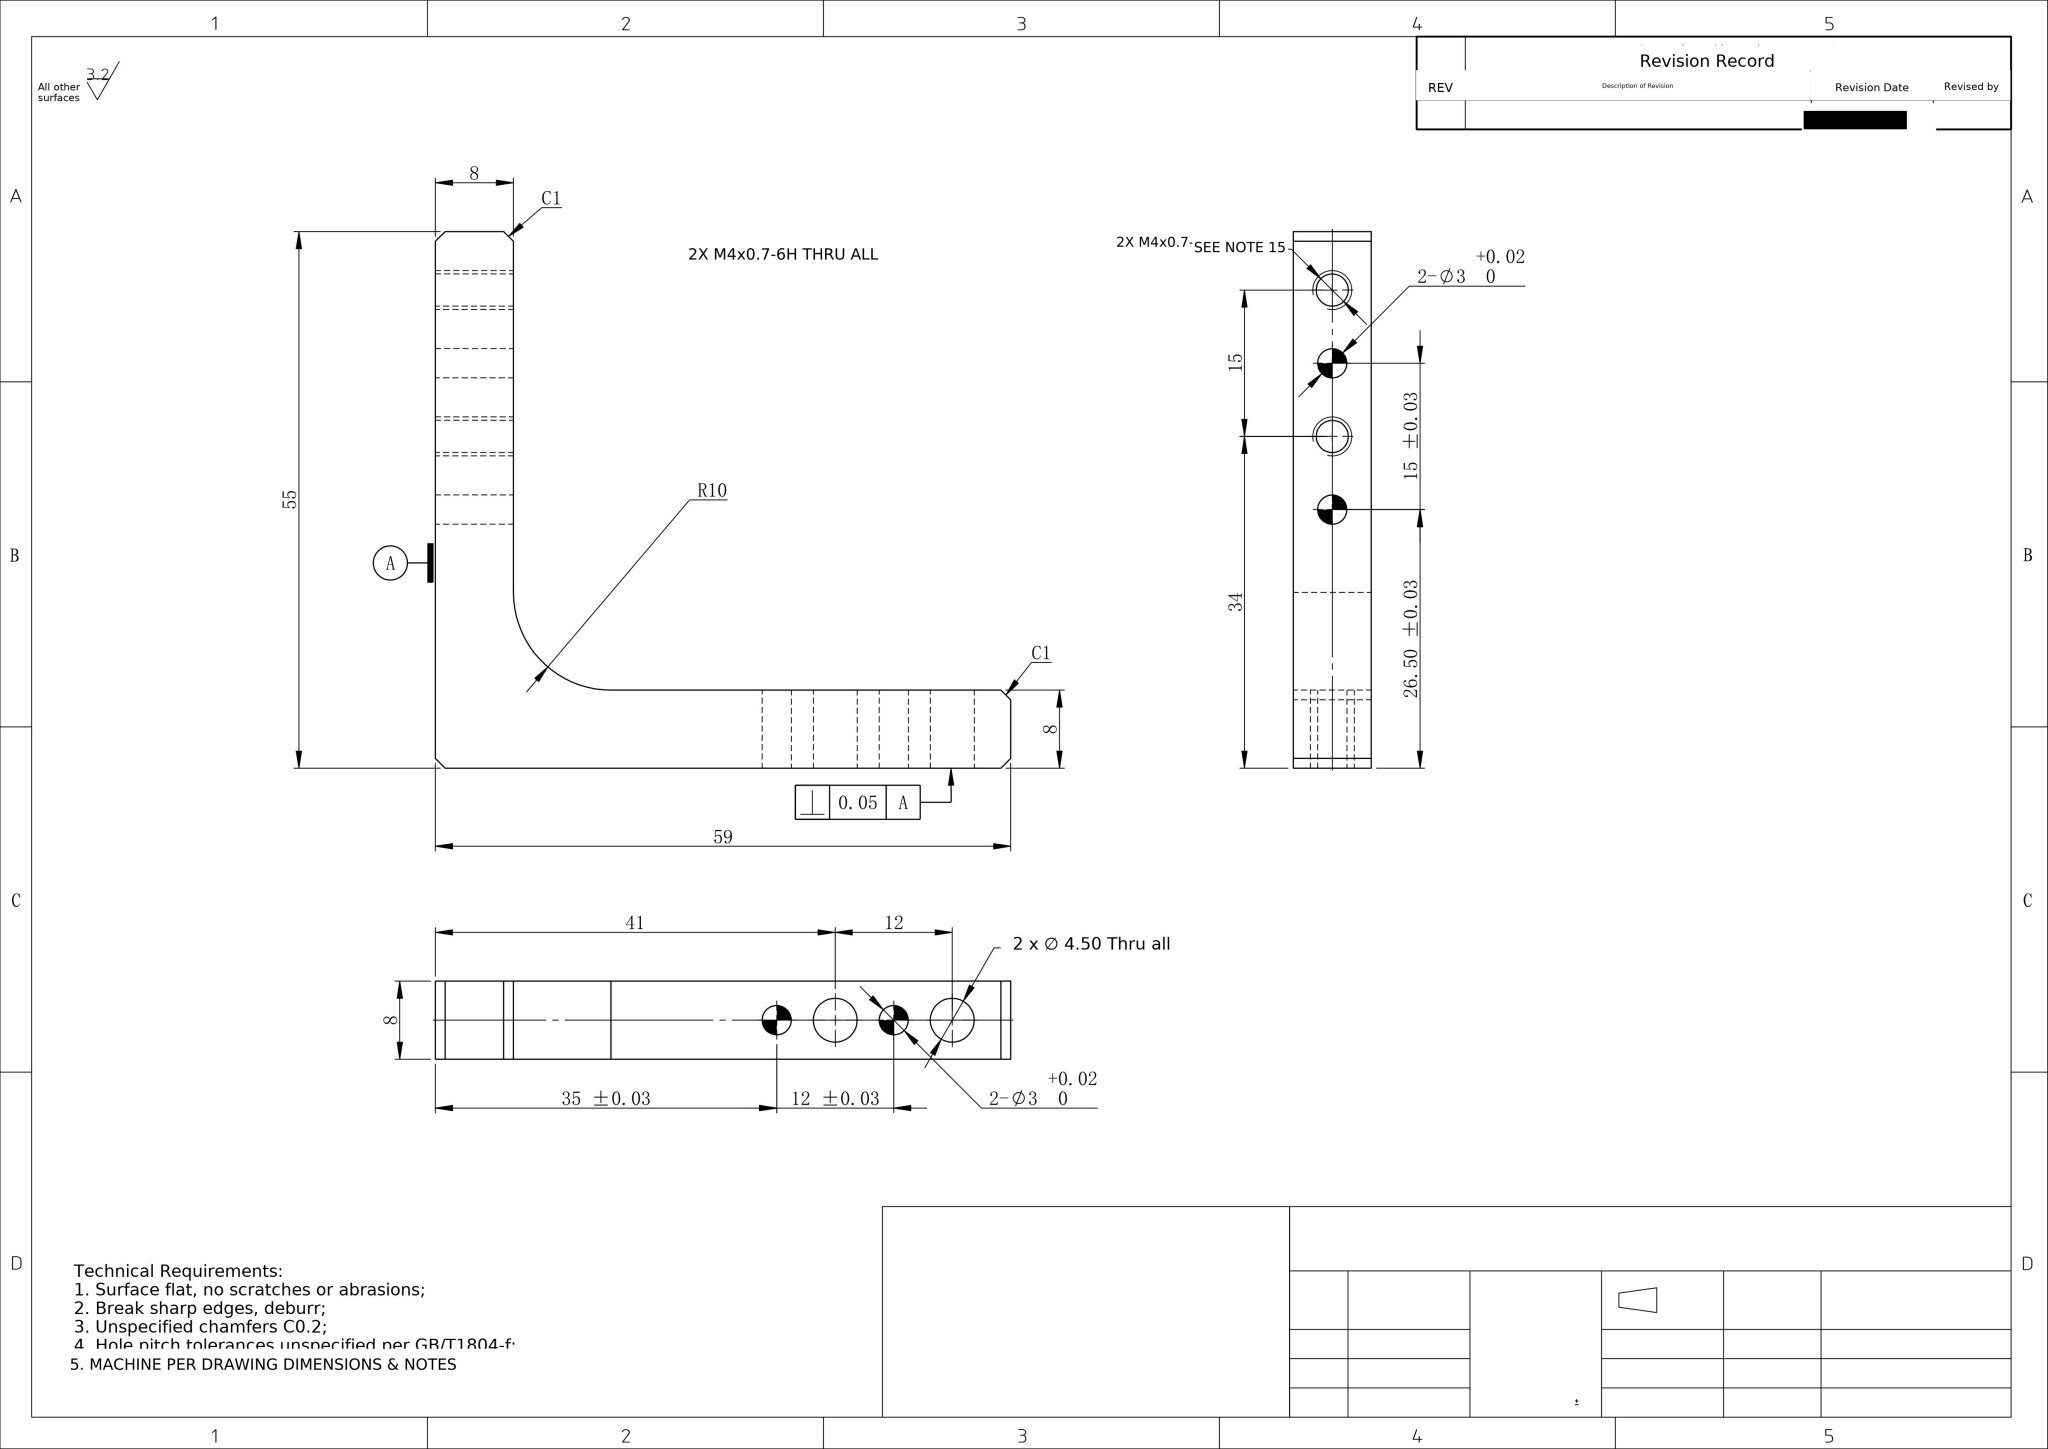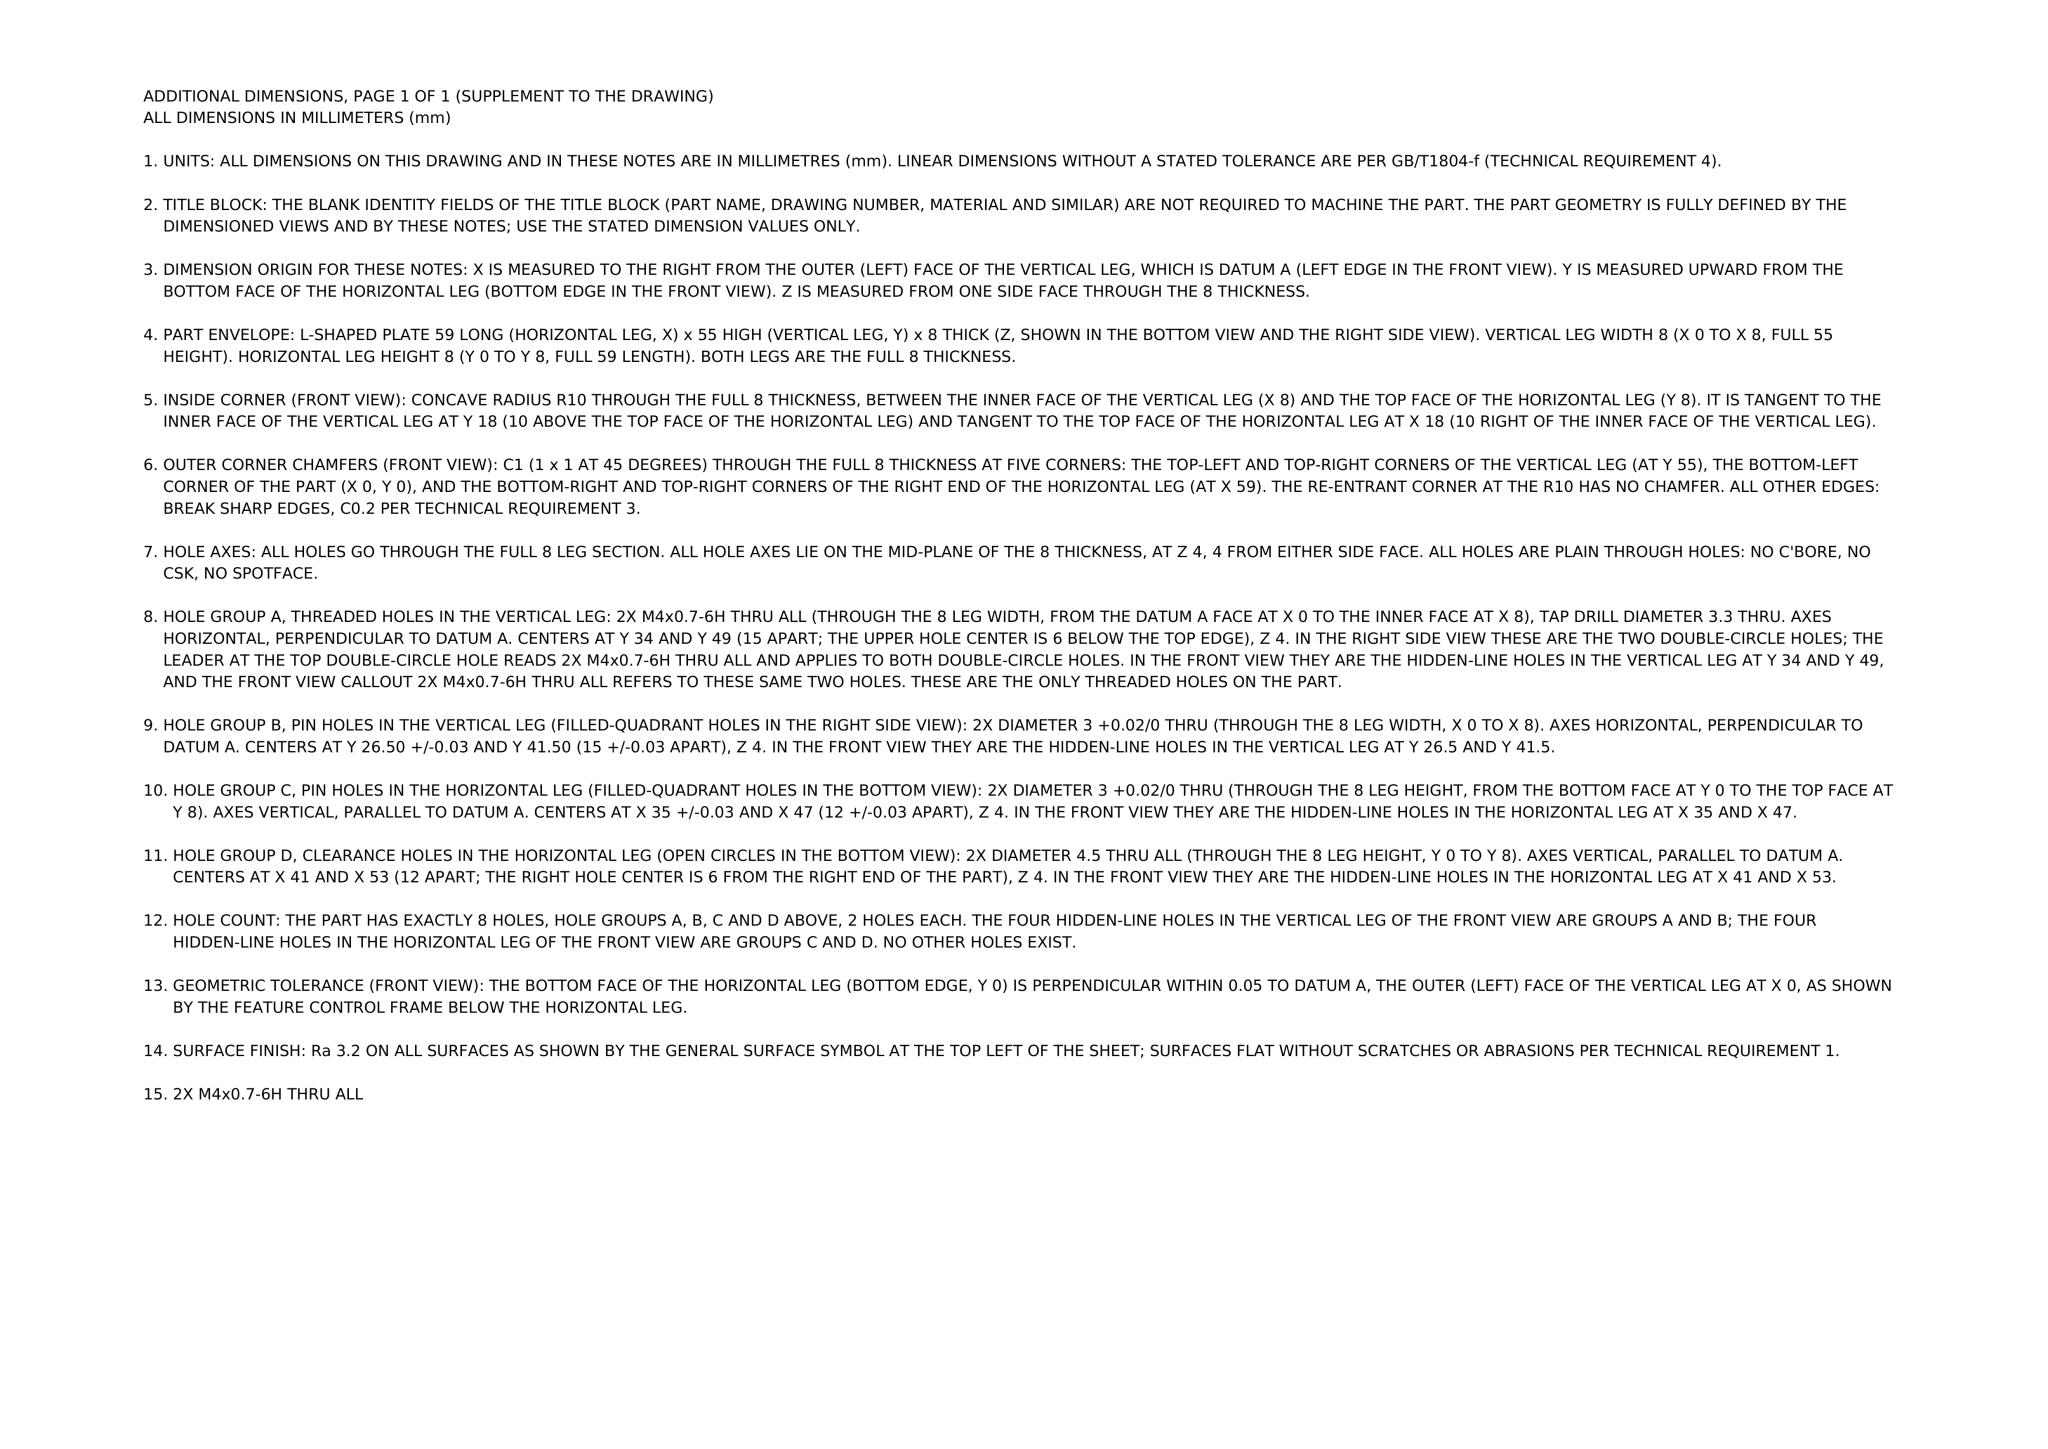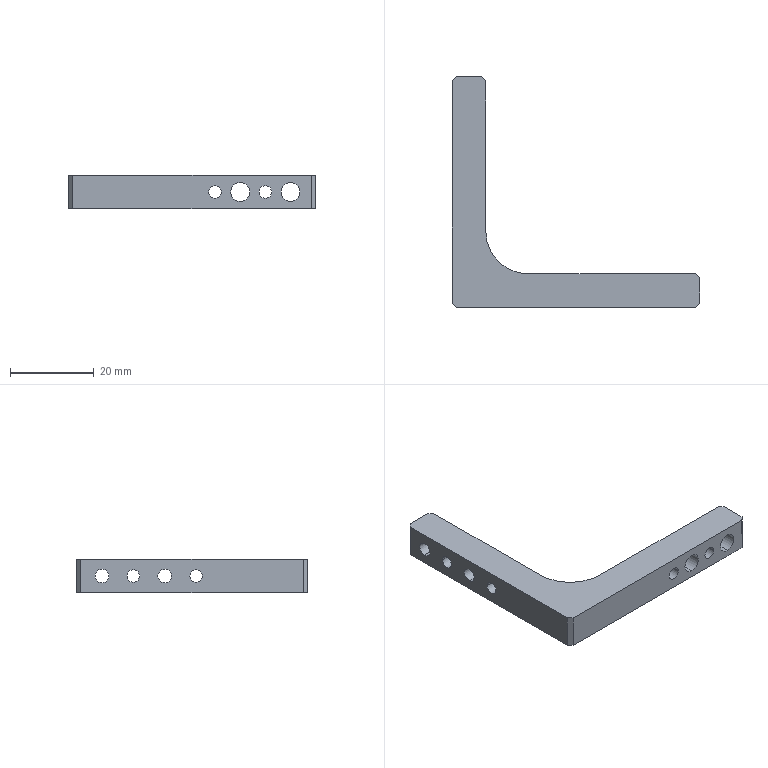Part | NX | mm | 1 solid | 30 faces | box 59 x 55 x 8 mm | volume 6318 mm3 | cylinder 17 | plane 13 | commonest cylinder face diameters 3 x8 3.3 x4 4.5 x4 20 x1